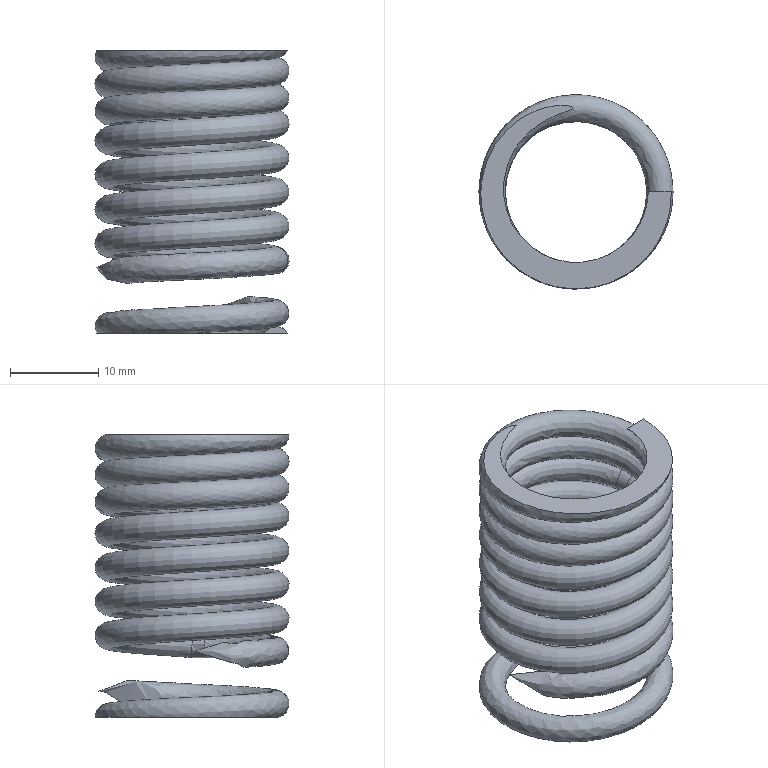Component | NX | SPRING_CYLINDER_COMPRESSION_1 | 1 solid | 9 faces | volume 3985 mm3 | spline 5 | plane 4